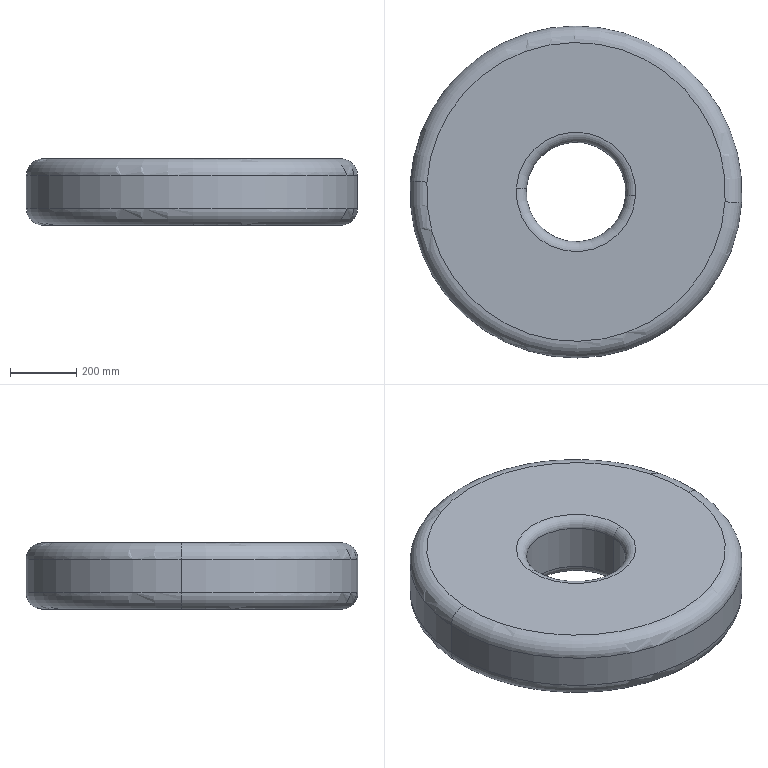Component | SolidWorks | RunningMechanism-4_9-17 | 1 solid | 14 faces | box 1000 x 1000 x 200 mm | volume 139266477 mm3 | torus 8 | cylinder 4 | plane 2 | commonest cylinder face diameters 300 x2 1000 x2
build123d program:
from build123d import *

# Parameters (mm, degrees)
SKETCH1_R           = 500
SKETCH1_R_2         = 150
BOSS_EXTRUDE1_DEPTH = 100
FILLET1_R           = 50
FILLET2_R           = 30


with BuildPart() as part:
    # Sketch1 → Boss-Extrude1 (new, symmetric)
    with BuildSketch(Plane.XY):
        Circle(SKETCH1_R)
        Circle(SKETCH1_R_2, mode=Mode.SUBTRACT)
    extrude(amount=BOSS_EXTRUDE1_DEPTH, both=True)

    # Fillet1
    fillet1_edges = [part.edges().sort_by_distance(p)[0] for p in [
        (-500, 0, -100),
        (-500, 0, 100),
    ]]
    fillet(fillet1_edges, radius=FILLET1_R)

    # Fillet2
    fillet2_edges = [part.edges().sort_by_distance(p)[0] for p in [
        (-150, 0, -100),
        (-150, 0, 100),
    ]]
    fillet(fillet2_edges, radius=FILLET2_R)


solid = part.part

# Placed as in the assembly
solid = solid.moved(Location((-8158.959, 55398.441, 24423.005), (0, 0, 0)))
STEP:
#1=CARTESIAN_POINT('',(-314.148,2180.574,965.473));
#2=VERTEX_POINT('',#1);
#3=CARTESIAN_POINT('',(-328.29,2181.508,965.473));
#4=VERTEX_POINT('',#3);
#5=CARTESIAN_POINT('',(-321.219,2181.041,965.473));
#6=DIRECTION('',(-0.0000002,0.,-1.));
#7=DIRECTION('',(-0.9978,0.06594,0.0000002));
#8=AXIS2_PLACEMENT_3D('',#5,#6,#7);
#9=CIRCLE('',#8,7.087);
#10=EDGE_CURVE('',#2,#4,#9,.T.);
#11=ORIENTED_EDGE('',*,*,#10,.F.);
#12=CARTESIAN_POINT('',(-315.326,2180.652,964.292));
#13=VERTEX_POINT('',#12);
#14=CARTESIAN_POINT('',(-314.148,2180.574,964.292));
#15=DIRECTION('',(-0.06594,-0.9978,0.00000001));
#16=DIRECTION('',(0.9978,-0.06594,0.));
#17=AXIS2_PLACEMENT_3D('',#14,#15,#16);
#18=CIRCLE('',#17,1.181);
#19=EDGE_CURVE('',#2,#13,#18,.T.);
#20=ORIENTED_EDGE('',*,*,#19,.T.);
#21=CARTESIAN_POINT('',(-327.112,2181.43,964.292));
#22=VERTEX_POINT('',#21);
#23=CARTESIAN_POINT('',(-321.219,2181.041,964.292));
#24=DIRECTION('',(0.0000002,-0.,1.));
#25=DIRECTION('',(-0.9978,0.06594,0.0000002));
#26=AXIS2_PLACEMENT_3D('',#23,#24,#25);
#27=CIRCLE('',#26,5.906);
#28=EDGE_CURVE('',#22,#13,#27,.T.);
#29=ORIENTED_EDGE('',*,*,#28,.F.);
#30=CARTESIAN_POINT('',(-328.29,2181.508,964.292));
#31=DIRECTION('',(0.06594,0.9978,-0.00000001));
#32=DIRECTION('',(-0.9978,0.06594,0.));
#33=AXIS2_PLACEMENT_3D('',#30,#31,#32);
#34=CIRCLE('',#33,1.181);
#35=EDGE_CURVE('',#4,#22,#34,.T.);
#36=ORIENTED_EDGE('',*,*,#35,.F.);
#37=EDGE_LOOP('',(#11,#20,#29,#36));
#38=FACE_OUTER_BOUND('',#37,.T.);
#39=CARTESIAN_POINT('',(-321.219,2181.041,964.292));
#40=DIRECTION('',(0.0000002,-0.,1.));
#41=DIRECTION('',(-0.9978,0.06594,0.0000002));
#42=AXIS2_PLACEMENT_3D('',#39,#40,#41);
#43=TOROIDAL_SURFACE('',#42,7.087,1.181);
#44=ADVANCED_FACE('',(#38),#43,.T.);
#45=CARTESIAN_POINT('',(-315.326,2180.652,958.78));
#46=VERTEX_POINT('',#45);
#47=CARTESIAN_POINT('',(-327.112,2181.43,958.78));
#48=VERTEX_POINT('',#47);
#49=CARTESIAN_POINT('',(-321.219,2181.041,958.78));
#50=DIRECTION('',(-0.0000002,0.,-1.));
#51=DIRECTION('',(-0.9978,0.06594,0.0000002));
#52=AXIS2_PLACEMENT_3D('',#49,#50,#51);
#53=CIRCLE('',#52,5.906);
#54=EDGE_CURVE('',#46,#48,#53,.T.);
#55=ORIENTED_EDGE('',*,*,#54,.F.);
#56=CARTESIAN_POINT('',(-314.148,2180.574,957.599));
#57=VERTEX_POINT('',#56);
#58=CARTESIAN_POINT('',(-314.148,2180.574,958.78));
#59=DIRECTION('',(-0.06594,-0.9978,0.00000001));
#60=DIRECTION('',(0.9978,-0.06594,0.));
#61=AXIS2_PLACEMENT_3D('',#58,#59,#60);
#62=CIRCLE('',#61,1.181);
#63=EDGE_CURVE('',#46,#57,#62,.T.);
#64=ORIENTED_EDGE('',*,*,#63,.T.);
#65=CARTESIAN_POINT('',(-328.29,2181.508,957.599));
#66=VERTEX_POINT('',#65);
#67=CARTESIAN_POINT('',(-321.219,2181.041,957.599));
#68=DIRECTION('',(0.0000002,-0.,1.));
#69=DIRECTION('',(-0.9978,0.06594,0.0000002));
#70=AXIS2_PLACEMENT_3D('',#67,#68,#69);
#71=CIRCLE('',#70,7.087);
#72=EDGE_CURVE('',#66,#57,#71,.T.);
#73=ORIENTED_EDGE('',*,*,#72,.F.);
#74=CARTESIAN_POINT('',(-328.29,2181.508,958.78));
#75=DIRECTION('',(0.06594,0.9978,-0.00000001));
#76=DIRECTION('',(-0.9978,0.06594,0.));
#77=AXIS2_PLACEMENT_3D('',#74,#75,#76);
#78=CIRCLE('',#77,1.181);
#79=EDGE_CURVE('',#48,#66,#78,.T.);
#80=ORIENTED_EDGE('',*,*,#79,.F.);
#81=EDGE_LOOP('',(#55,#64,#73,#80));
#82=FACE_OUTER_BOUND('',#81,.T.);
#83=CARTESIAN_POINT('',(-321.219,2181.041,958.78));
#84=DIRECTION('',(0.0000002,-0.,1.));
#85=DIRECTION('',(-0.9978,0.06594,0.0000002));
#86=AXIS2_PLACEMENT_3D('',#83,#84,#85);
#87=TOROIDAL_SURFACE('',#86,7.087,1.181);
#88=ADVANCED_FACE('',(#82),#87,.T.);
#89=CARTESIAN_POINT('',(-301.577,2179.743,963.504));
#90=VERTEX_POINT('',#89);
#91=CARTESIAN_POINT('',(-340.861,2182.339,963.504));
#92=VERTEX_POINT('',#91);
#93=CARTESIAN_POINT('',(-321.219,2181.041,963.504));
#94=DIRECTION('',(-0.0000002,0.,-1.));
#95=DIRECTION('',(-0.9978,0.06594,0.0000002));
#96=AXIS2_PLACEMENT_3D('',#93,#94,#95);
#97=CIRCLE('',#96,19.685);
#98=EDGE_CURVE('',#90,#92,#97,.T.);
#99=ORIENTED_EDGE('',*,*,#98,.F.);
#100=CARTESIAN_POINT('',(-303.541,2179.873,965.473));
#101=VERTEX_POINT('',#100);
#102=CARTESIAN_POINT('',(-303.541,2179.873,963.504));
#103=DIRECTION('',(-0.06594,-0.9978,0.00000001));
#104=DIRECTION('',(0.9978,-0.06594,0.));
#105=AXIS2_PLACEMENT_3D('',#102,#103,#104);
#106=CIRCLE('',#105,1.969);
#107=EDGE_CURVE('',#90,#101,#106,.T.);
#108=ORIENTED_EDGE('',*,*,#107,.T.);
#109=CARTESIAN_POINT('',(-338.897,2182.209,965.473));
#110=VERTEX_POINT('',#109);
#111=CARTESIAN_POINT('',(-321.219,2181.041,965.473));
#112=DIRECTION('',(0.0000002,-0.,1.));
#113=DIRECTION('',(-0.9978,0.06594,0.0000002));
#114=AXIS2_PLACEMENT_3D('',#111,#112,#113);
#115=CIRCLE('',#114,17.717);
#116=EDGE_CURVE('',#110,#101,#115,.T.);
#117=ORIENTED_EDGE('',*,*,#116,.F.);
#118=CARTESIAN_POINT('',(-338.897,2182.209,963.504));
#119=DIRECTION('',(0.06594,0.9978,-0.00000001));
#120=DIRECTION('',(-0.9978,0.06594,0.));
#121=AXIS2_PLACEMENT_3D('',#118,#119,#120);
#122=CIRCLE('',#121,1.969);
#123=EDGE_CURVE('',#92,#110,#122,.T.);
#124=ORIENTED_EDGE('',*,*,#123,.F.);
#125=EDGE_LOOP('',(#99,#108,#117,#124));
#126=FACE_OUTER_BOUND('',#125,.T.);
#127=CARTESIAN_POINT('',(-321.219,2181.041,963.504));
#128=DIRECTION('',(0.0000002,-0.,1.));
#129=DIRECTION('',(-0.9978,0.06594,0.0000002));
#130=AXIS2_PLACEMENT_3D('',#127,#128,#129);
#131=TOROIDAL_SURFACE('',#130,17.717,1.969);
#132=ADVANCED_FACE('',(#126),#131,.T.);
#133=CARTESIAN_POINT('',(-303.541,2179.873,957.599));
#134=VERTEX_POINT('',#133);
#135=CARTESIAN_POINT('',(-338.897,2182.209,957.599));
#136=VERTEX_POINT('',#135);
#137=CARTESIAN_POINT('',(-321.219,2181.041,957.599));
#138=DIRECTION('',(-0.0000002,0.,-1.));
#139=DIRECTION('',(-0.9978,0.06594,0.0000002));
#140=AXIS2_PLACEMENT_3D('',#137,#138,#139);
#141=CIRCLE('',#140,17.717);
#142=EDGE_CURVE('',#134,#136,#141,.T.);
#143=ORIENTED_EDGE('',*,*,#142,.F.);
#144=CARTESIAN_POINT('',(-301.577,2179.743,959.567));
#145=VERTEX_POINT('',#144);
#146=CARTESIAN_POINT('',(-303.541,2179.873,959.567));
#147=DIRECTION('',(-0.06594,-0.9978,0.00000001));
#148=DIRECTION('',(0.9978,-0.06594,0.));
#149=AXIS2_PLACEMENT_3D('',#146,#147,#148);
#150=CIRCLE('',#149,1.969);
#151=EDGE_CURVE('',#134,#145,#150,.T.);
#152=ORIENTED_EDGE('',*,*,#151,.T.);
#153=CARTESIAN_POINT('',(-340.861,2182.339,959.567));
#154=VERTEX_POINT('',#153);
#155=CARTESIAN_POINT('',(-321.219,2181.041,959.567));
#156=DIRECTION('',(0.0000002,-0.,1.));
#157=DIRECTION('',(-0.9978,0.06594,0.0000002));
#158=AXIS2_PLACEMENT_3D('',#155,#156,#157);
#159=CIRCLE('',#158,19.685);
#160=EDGE_CURVE('',#154,#145,#159,.T.);
#161=ORIENTED_EDGE('',*,*,#160,.F.);
#162=CARTESIAN_POINT('',(-338.897,2182.209,959.567));
#163=DIRECTION('',(0.06594,0.9978,-0.00000001));
#164=DIRECTION('',(-0.9978,0.06594,0.));
#165=AXIS2_PLACEMENT_3D('',#162,#163,#164);
#166=CIRCLE('',#165,1.969);
#167=EDGE_CURVE('',#136,#154,#166,.T.);
#168=ORIENTED_EDGE('',*,*,#167,.F.);
#169=EDGE_LOOP('',(#143,#152,#161,#168));
#170=FACE_OUTER_BOUND('',#169,.T.);
#171=CARTESIAN_POINT('',(-321.219,2181.041,959.567));
#172=DIRECTION('',(0.0000002,-0.,1.));
#173=DIRECTION('',(-0.9978,0.06594,0.0000002));
#174=AXIS2_PLACEMENT_3D('',#171,#172,#173);
#175=TOROIDAL_SURFACE('',#174,17.717,1.969);
#176=ADVANCED_FACE('',(#170),#175,.T.);
#177=CARTESIAN_POINT('',(-321.219,2181.041,964.292));
#178=DIRECTION('',(0.0000002,-0.,1.));
#179=DIRECTION('',(-0.9978,0.06594,0.0000002));
#180=AXIS2_PLACEMENT_3D('',#177,#178,#179);
#181=CIRCLE('',#180,5.906);
#182=EDGE_CURVE('',#13,#22,#181,.T.);
#183=ORIENTED_EDGE('',*,*,#182,.T.);
#184=CARTESIAN_POINT('',(-327.112,2181.43,965.473));
#185=DIRECTION('',(-0.0000002,0.,-1.));
#186=VECTOR('',#185,39.37);
#187=LINE('',#184,#186);
#188=EDGE_CURVE('',#22,#48,#187,.T.);
#189=ORIENTED_EDGE('',*,*,#188,.T.);
#190=CARTESIAN_POINT('',(-321.219,2181.041,958.78));
#191=DIRECTION('',(-0.0000002,0.,-1.));
#192=DIRECTION('',(-0.9978,0.06594,0.0000002));
#193=AXIS2_PLACEMENT_3D('',#190,#191,#192);
#194=CIRCLE('',#193,5.906);
#195=EDGE_CURVE('',#48,#46,#194,.T.);
#196=ORIENTED_EDGE('',*,*,#195,.T.);
#197=CARTESIAN_POINT('',(-315.326,2180.652,965.473));
#198=DIRECTION('',(-0.0000002,0.,-1.));
#199=VECTOR('',#198,39.37);
#200=LINE('',#197,#199);
#201=EDGE_CURVE('',#13,#46,#200,.T.);
#202=ORIENTED_EDGE('',*,*,#201,.F.);
#203=EDGE_LOOP('',(#183,#189,#196,#202));
#204=FACE_OUTER_BOUND('',#203,.T.);
#205=CARTESIAN_POINT('',(-321.219,2181.041,965.473));
#206=DIRECTION('',(-0.0000002,0.,-1.));
#207=DIRECTION('',(0.9978,-0.06594,-0.0000002));
#208=AXIS2_PLACEMENT_3D('',#205,#206,#207);
#209=CYLINDRICAL_SURFACE('',#208,5.906);
#210=ADVANCED_FACE('',(#204),#209,.F.);
#211=ORIENTED_EDGE('',*,*,#98,.T.);
#212=CARTESIAN_POINT('',(-340.861,2182.339,965.473));
#213=DIRECTION('',(-0.0000002,0.,-1.));
#214=VECTOR('',#213,39.37);
#215=LINE('',#212,#214);
#216=EDGE_CURVE('',#92,#154,#215,.T.);
#217=ORIENTED_EDGE('',*,*,#216,.T.);
#218=ORIENTED_EDGE('',*,*,#160,.T.);
#219=CARTESIAN_POINT('',(-301.577,2179.743,965.473));
#220=DIRECTION('',(-0.0000002,0.,-1.));
#221=VECTOR('',#220,39.37);
#222=LINE('',#219,#221);
#223=EDGE_CURVE('',#90,#145,#222,.T.);
#224=ORIENTED_EDGE('',*,*,#223,.F.);
#225=EDGE_LOOP('',(#211,#217,#218,#224));
#226=FACE_OUTER_BOUND('',#225,.T.);
#227=CARTESIAN_POINT('',(-321.219,2181.041,965.473));
#228=DIRECTION('',(-0.0000002,0.,-1.));
#229=DIRECTION('',(0.9978,-0.06594,-0.0000002));
#230=AXIS2_PLACEMENT_3D('',#227,#228,#229);
#231=CYLINDRICAL_SURFACE('',#230,19.685);
#232=ADVANCED_FACE('',(#226),#231,.T.);
#233=CARTESIAN_POINT('',(-321.219,2181.041,965.473));
#234=DIRECTION('',(-0.0000002,0.,-1.));
#235=DIRECTION('',(-0.9978,0.06594,0.0000002));
#236=AXIS2_PLACEMENT_3D('',#233,#234,#235);
#237=CIRCLE('',#236,7.087);
#238=EDGE_CURVE('',#4,#2,#237,.T.);
#239=ORIENTED_EDGE('',*,*,#238,.T.);
#240=ORIENTED_EDGE('',*,*,#10,.T.);
#241=EDGE_LOOP('',(#239,#240));
#242=FACE_BOUND('',#241,.T.);
#243=ORIENTED_EDGE('',*,*,#116,.T.);
#244=CARTESIAN_POINT('',(-321.219,2181.041,965.473));
#245=DIRECTION('',(0.0000002,-0.,1.));
#246=DIRECTION('',(-0.9978,0.06594,0.0000002));
#247=AXIS2_PLACEMENT_3D('',#244,#245,#246);
#248=CIRCLE('',#247,17.717);
#249=EDGE_CURVE('',#101,#110,#248,.T.);
#250=ORIENTED_EDGE('',*,*,#249,.T.);
#251=EDGE_LOOP('',(#243,#250));
#252=FACE_OUTER_BOUND('',#251,.T.);
#253=CARTESIAN_POINT('',(-321.219,2181.041,965.473));
#254=DIRECTION('',(0.0000002,-0.,1.));
#255=DIRECTION('',(-0.9978,0.06594,0.0000002));
#256=AXIS2_PLACEMENT_3D('',#253,#254,#255);
#257=PLANE('',#256);
#258=ADVANCED_FACE('',(#242,#252),#257,.T.);
#259=ORIENTED_EDGE('',*,*,#72,.T.);
#260=CARTESIAN_POINT('',(-321.219,2181.041,957.599));
#261=DIRECTION('',(0.0000002,-0.,1.));
#262=DIRECTION('',(-0.9978,0.06594,0.0000002));
#263=AXIS2_PLACEMENT_3D('',#260,#261,#262);
#264=CIRCLE('',#263,7.087);
#265=EDGE_CURVE('',#57,#66,#264,.T.);
#266=ORIENTED_EDGE('',*,*,#265,.T.);
#267=EDGE_LOOP('',(#259,#266));
#268=FACE_BOUND('',#267,.T.);
#269=CARTESIAN_POINT('',(-321.219,2181.041,957.599));
#270=DIRECTION('',(-0.0000002,0.,-1.));
#271=DIRECTION('',(-0.9978,0.06594,0.0000002));
#272=AXIS2_PLACEMENT_3D('',#269,#270,#271);
#273=CIRCLE('',#272,17.717);
#274=EDGE_CURVE('',#136,#134,#273,.T.);
#275=ORIENTED_EDGE('',*,*,#274,.T.);
#276=ORIENTED_EDGE('',*,*,#142,.T.);
#277=EDGE_LOOP('',(#275,#276));
#278=FACE_OUTER_BOUND('',#277,.T.);
#279=CARTESIAN_POINT('',(-321.219,2181.041,957.599));
#280=DIRECTION('',(0.0000002,-0.,1.));
#281=DIRECTION('',(-0.9978,0.06594,0.0000002));
#282=AXIS2_PLACEMENT_3D('',#279,#280,#281);
#283=PLANE('',#282);
#284=ADVANCED_FACE('',(#268,#278),#283,.F.);
#285=ORIENTED_EDGE('',*,*,#216,.F.);
#286=CARTESIAN_POINT('',(-321.219,2181.041,963.504));
#287=DIRECTION('',(-0.0000002,0.,-1.));
#288=DIRECTION('',(-0.9978,0.06594,0.0000002));
#289=AXIS2_PLACEMENT_3D('',#286,#287,#288);
#290=CIRCLE('',#289,19.685);
#291=EDGE_CURVE('',#92,#90,#290,.T.);
#292=ORIENTED_EDGE('',*,*,#291,.T.);
#293=ORIENTED_EDGE('',*,*,#223,.T.);
#294=CARTESIAN_POINT('',(-321.219,2181.041,959.567));
#295=DIRECTION('',(0.0000002,-0.,1.));
#296=DIRECTION('',(-0.9978,0.06594,0.0000002));
#297=AXIS2_PLACEMENT_3D('',#294,#295,#296);
#298=CIRCLE('',#297,19.685);
#299=EDGE_CURVE('',#145,#154,#298,.T.);
#300=ORIENTED_EDGE('',*,*,#299,.T.);
#301=EDGE_LOOP('',(#285,#292,#293,#300));
#302=FACE_OUTER_BOUND('',#301,.T.);
#303=CARTESIAN_POINT('',(-321.219,2181.041,965.473));
#304=DIRECTION('',(-0.0000002,0.,-1.));
#305=DIRECTION('',(0.9978,-0.06594,-0.0000002));
#306=AXIS2_PLACEMENT_3D('',#303,#304,#305);
#307=CYLINDRICAL_SURFACE('',#306,19.685);
#308=ADVANCED_FACE('',(#302),#307,.T.);
#309=ORIENTED_EDGE('',*,*,#188,.F.);
#310=ORIENTED_EDGE('',*,*,#28,.T.);
#311=ORIENTED_EDGE('',*,*,#201,.T.);
#312=ORIENTED_EDGE('',*,*,#54,.T.);
#313=EDGE_LOOP('',(#309,#310,#311,#312));
#314=FACE_OUTER_BOUND('',#313,.T.);
#315=CARTESIAN_POINT('',(-321.219,2181.041,965.473));
#316=DIRECTION('',(-0.0000002,0.,-1.));
#317=DIRECTION('',(0.9978,-0.06594,-0.0000002));
#318=AXIS2_PLACEMENT_3D('',#315,#316,#317);
#319=CYLINDRICAL_SURFACE('',#318,5.906);
#320=ADVANCED_FACE('',(#314),#319,.F.);
#321=ORIENTED_EDGE('',*,*,#151,.F.);
#322=ORIENTED_EDGE('',*,*,#274,.F.);
#323=ORIENTED_EDGE('',*,*,#167,.T.);
#324=ORIENTED_EDGE('',*,*,#299,.F.);
#325=EDGE_LOOP('',(#321,#322,#323,#324));
#326=FACE_OUTER_BOUND('',#325,.T.);
#327=CARTESIAN_POINT('',(-321.219,2181.041,959.567));
#328=DIRECTION('',(0.0000002,-0.,1.));
#329=DIRECTION('',(-0.9978,0.06594,0.0000002));
#330=AXIS2_PLACEMENT_3D('',#327,#328,#329);
#331=TOROIDAL_SURFACE('',#330,17.717,1.969);
#332=ADVANCED_FACE('',(#326),#331,.T.);
#333=ORIENTED_EDGE('',*,*,#107,.F.);
#334=ORIENTED_EDGE('',*,*,#291,.F.);
#335=ORIENTED_EDGE('',*,*,#123,.T.);
#336=ORIENTED_EDGE('',*,*,#249,.F.);
#337=EDGE_LOOP('',(#333,#334,#335,#336));
#338=FACE_OUTER_BOUND('',#337,.T.);
#339=CARTESIAN_POINT('',(-321.219,2181.041,963.504));
#340=DIRECTION('',(0.0000002,-0.,1.));
#341=DIRECTION('',(-0.9978,0.06594,0.0000002));
#342=AXIS2_PLACEMENT_3D('',#339,#340,#341);
#343=TOROIDAL_SURFACE('',#342,17.717,1.969);
#344=ADVANCED_FACE('',(#338),#343,.T.);
#345=ORIENTED_EDGE('',*,*,#63,.F.);
#346=ORIENTED_EDGE('',*,*,#195,.F.);
#347=ORIENTED_EDGE('',*,*,#79,.T.);
#348=ORIENTED_EDGE('',*,*,#265,.F.);
#349=EDGE_LOOP('',(#345,#346,#347,#348));
#350=FACE_OUTER_BOUND('',#349,.T.);
#351=CARTESIAN_POINT('',(-321.219,2181.041,958.78));
#352=DIRECTION('',(0.0000002,-0.,1.));
#353=DIRECTION('',(-0.9978,0.06594,0.0000002));
#354=AXIS2_PLACEMENT_3D('',#351,#352,#353);
#355=TOROIDAL_SURFACE('',#354,7.087,1.181);
#356=ADVANCED_FACE('',(#350),#355,.T.);
#357=ORIENTED_EDGE('',*,*,#19,.F.);
#358=ORIENTED_EDGE('',*,*,#238,.F.);
#359=ORIENTED_EDGE('',*,*,#35,.T.);
#360=ORIENTED_EDGE('',*,*,#182,.F.);
#361=EDGE_LOOP('',(#357,#358,#359,#360));
#362=FACE_OUTER_BOUND('',#361,.T.);
#363=CARTESIAN_POINT('',(-321.219,2181.041,964.292));
#364=DIRECTION('',(0.0000002,-0.,1.));
#365=DIRECTION('',(-0.9978,0.06594,0.0000002));
#366=AXIS2_PLACEMENT_3D('',#363,#364,#365);
#367=TOROIDAL_SURFACE('',#366,7.087,1.181);
#368=ADVANCED_FACE('',(#362),#367,.T.);
#369=CLOSED_SHELL('',(#44,#88,#132,#176,#210,#232,#258,#284,#308,#320,#332,#344,#356,#368));
#370=MANIFOLD_SOLID_BREP('',#369);
#371=CARTESIAN_POINT('',(0.,0.,0.));
#372=DIRECTION('',(0.,0.,1.));
#373=DIRECTION('',(1.,0.,0.));
#374=AXIS2_PLACEMENT_3D('',#371,#372,#373);
#375=(LENGTH_UNIT()NAMED_UNIT(*)SI_UNIT($,.METRE.));
#376=LENGTH_MEASURE_WITH_UNIT(LENGTH_MEASURE(0.0254),#375);
#377=DIMENSIONAL_EXPONENTS(1.,0.,0.,0.,0.,0.,0.);
#378=(CONVERSION_BASED_UNIT('',#376)LENGTH_UNIT()NAMED_UNIT(#377));
#379=UNCERTAINTY_MEASURE_WITH_UNIT(LENGTH_MEASURE(0.00001),#378,'','');
#380=(NAMED_UNIT(*)PLANE_ANGLE_UNIT()SI_UNIT($,.RADIAN.));
#381=(NAMED_UNIT(*)SI_UNIT($,.STERADIAN.)SOLID_ANGLE_UNIT());
#382=(GEOMETRIC_REPRESENTATION_CONTEXT(3)GLOBAL_UNCERTAINTY_ASSIGNED_CONTEXT((#379))GLOBAL_UNIT_ASSIGNED_CONTEXT((#378,#380,#381))REPRESENTATION_CONTEXT('',''));
#383=ADVANCED_BREP_SHAPE_REPRESENTATION('',(#370,#374),#382);
#384=COLOUR_RGB('',0.7922,0.8196,0.9333);
#385=FILL_AREA_STYLE_COLOUR('',#384);
#386=FILL_AREA_STYLE('',(#385));
#387=SURFACE_STYLE_FILL_AREA(#386);
#388=SURFACE_SIDE_STYLE('',(#387));
#389=SURFACE_STYLE_USAGE(.BOTH.,#388);
#390=PRESENTATION_STYLE_ASSIGNMENT((#389));
#391=STYLED_ITEM('',(#390),#370);
#392=PRESENTATION_LAYER_ASSIGNMENT('','',(#391));
#393=(LENGTH_UNIT()NAMED_UNIT(*)SI_UNIT($,.METRE.));
#394=LENGTH_MEASURE_WITH_UNIT(LENGTH_MEASURE(0.0254),#393);
#395=DIMENSIONAL_EXPONENTS(1.,0.,0.,0.,0.,0.,0.);
#396=(CONVERSION_BASED_UNIT('',#394)LENGTH_UNIT()NAMED_UNIT(#395));
#397=UNCERTAINTY_MEASURE_WITH_UNIT(LENGTH_MEASURE(0.00001),#396,'','');
#398=(NAMED_UNIT(*)PLANE_ANGLE_UNIT()SI_UNIT($,.RADIAN.));
#399=(NAMED_UNIT(*)SI_UNIT($,.STERADIAN.)SOLID_ANGLE_UNIT());
#400=(GEOMETRIC_REPRESENTATION_CONTEXT(3)GLOBAL_UNCERTAINTY_ASSIGNED_CONTEXT((#397))GLOBAL_UNIT_ASSIGNED_CONTEXT((#396,#398,#399))REPRESENTATION_CONTEXT('',''));
#401=MECHANICAL_DESIGN_GEOMETRIC_PRESENTATION_REPRESENTATION('',(#391),#400);